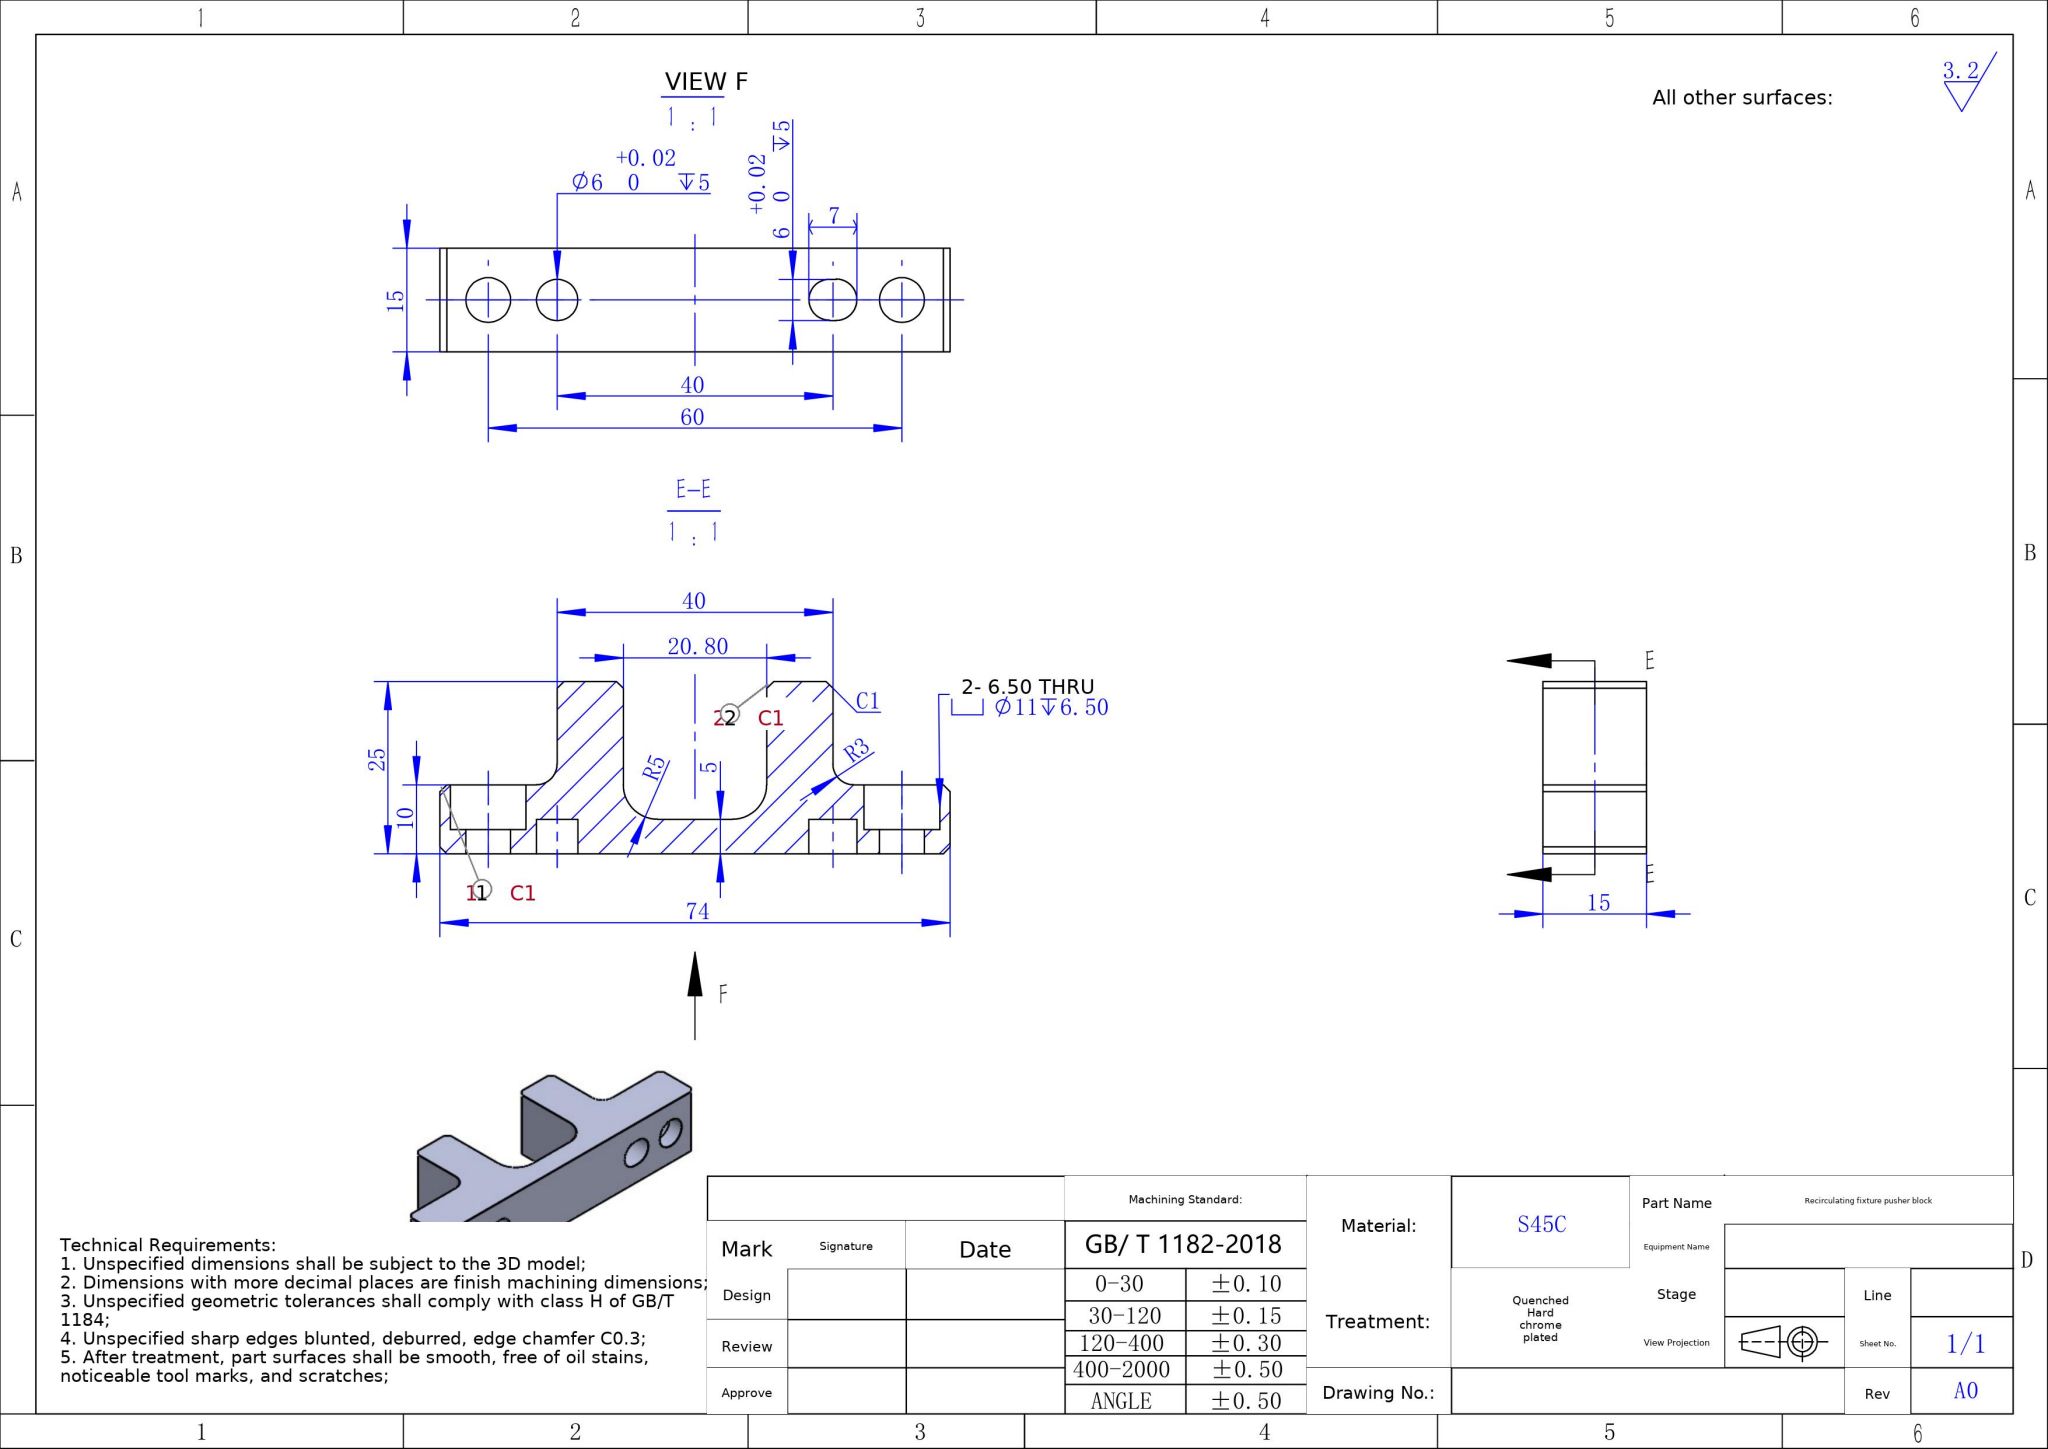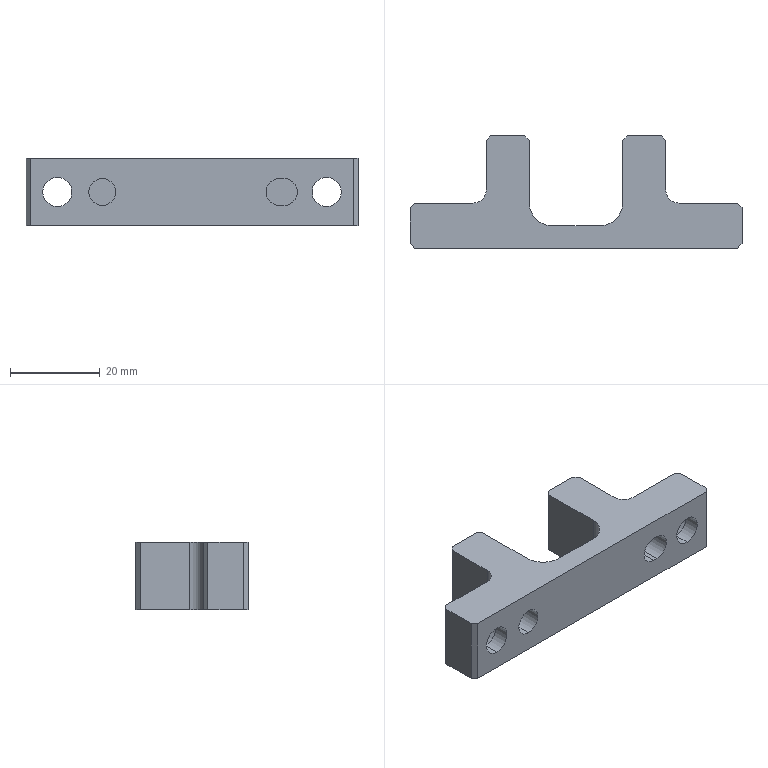Part | SolidWorks | mm | material S45C | 1 solid | 44 faces | box 74 x 25 x 15 mm | volume 12238 mm3 | plane 28 | cylinder 16 | commonest cylinder face diameters 6 x6 11 x4 6.5 x4 10 x2
build123d program:
from build123d import *

# Parameters (mm, degrees)
BOSS_EXTRUDE1_DEPTH = 7.5
FILLET1_R           = 5
CHAMFER1_SIZE       = 1
CHAMFER2_SIZE       = 1
SKETCH2_R           = 3.25
CUT_EXTRUDE1_DEPTH  = 15
SKETCH3_R           = 5.5
CUT_EXTRUDE2_DEPTH  = 6.5
SKETCH4_R           = 3
CUT_EXTRUDE3_DEPTH  = 5
FILLET2_R           = 3


with BuildPart() as part:
    # Sketch1 → Boss-Extrude1 (new, symmetric)
    with BuildSketch(Plane.XY):
        Polygon((-10.4, 0), (10.4, 0), (10.4, 20), (20, 20), (20, 5), (37, 5), (37, -5), (-37, -5), (-37, 5), (-20, 5), (-20, 20), (-10.4, 20), align=None)
    extrude(amount=BOSS_EXTRUDE1_DEPTH, both=True)

    # Fillet1
    fillet1_edges = [part.edges().sort_by_distance(p)[0] for p in [
        (-10.4, 0, 0),
        (10.4, 0, 0),
    ]]
    fillet(fillet1_edges, radius=FILLET1_R)

    # Chamfer1
    chamfer1_edges = [part.edges().sort_by_distance(p)[0] for p in [
        (10.4, 20, 0),
        (-10.4, 20, 0),
    ]]
    chamfer(chamfer1_edges, length=CHAMFER1_SIZE)

    # Chamfer2
    chamfer2_edges = [part.edges().sort_by_distance(p)[0] for p in [
        (20, 20, 0),
        (37, 5, 0),
        (37, -5, 0),
        (-37, -5, 0),
        (-37, 5, 0),
        (-20, 20, 0),
    ]]
    chamfer(chamfer2_edges, length=CHAMFER2_SIZE)

    # Sketch2 → Cut-Extrude1 (cut)
    with BuildSketch(Plane(origin=(0, 5, 0), x_dir=(1, 0, 0), z_dir=(0, 1, 0))):
        with Locations(Location((30, 0, 0), (0, 0, 270))):
            Circle(SKETCH2_R)
        with Locations(Location((-30, 0, 0), (0, 0, 270))):
            Circle(SKETCH2_R)
    extrude(amount=-CUT_EXTRUDE1_DEPTH, mode=Mode.SUBTRACT)

    # Sketch3 → Cut-Extrude2 (cut)
    with BuildSketch(Plane(origin=(0, 5, 0), x_dir=(1, 0, 0), z_dir=(0, 1, 0))):
        with Locations(Location((30, 0, 0), (0, 0, 270))):
            Circle(SKETCH3_R)
        with Locations(Location((-30, 0, 0), (0, 0, 270))):
            Circle(SKETCH3_R)
    extrude(amount=-CUT_EXTRUDE2_DEPTH, mode=Mode.SUBTRACT)

    # Sketch4 → Cut-Extrude3 (cut)
    with BuildSketch(Plane.XZ.offset(5)):
        with Locations(Location((-20, 0, 0), (0, 0, 270))):
            Circle(SKETCH4_R)
        with BuildLine():
            Line((19.5, 3), (20.5, 3))
            ThreePointArc((20.5, 3), (23.5, 0), (20.5, -3))
            Line((20.5, -3), (19.5, -3))
            ThreePointArc((19.5, -3), (16.5, 0), (19.5, 3))
        make_face()
    extrude(amount=-CUT_EXTRUDE3_DEPTH, mode=Mode.SUBTRACT)

    # Fillet2
    fillet2_edges = [part.edges().sort_by_distance(p)[0] for p in [
        (20, 5, 0),
        (-20, 5, 0),
    ]]
    fillet(fillet2_edges, radius=FILLET2_R)


solid = part.part